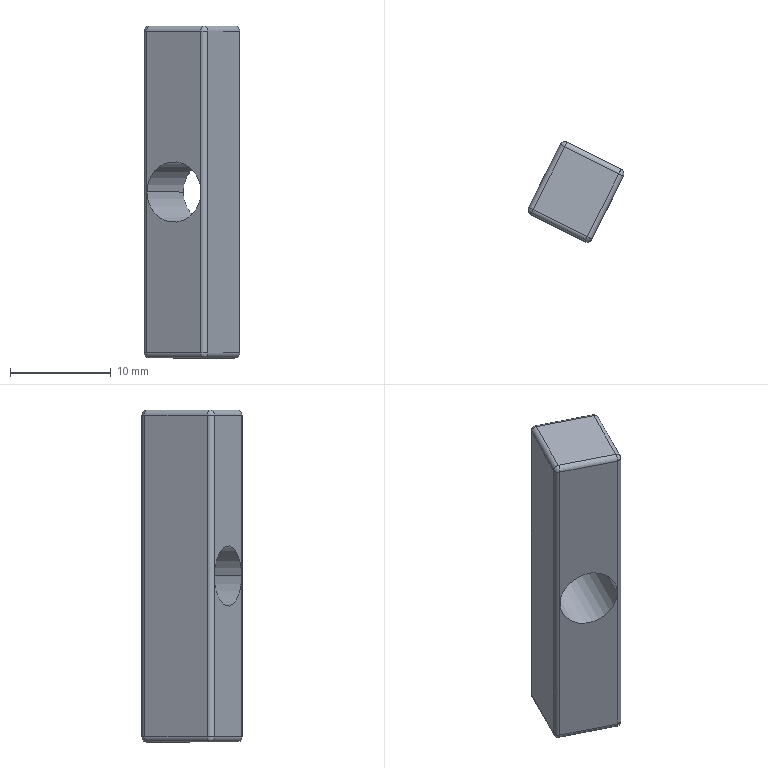Component | SolidWorks | ConnectingBlock1-1 | 1 solid | 29 faces | box 9.52 x 9.96 x 33 mm | volume 1616 mm3 | cylinder 15 | sphere 8 | plane 6 | commonest cylinder face diameters 1 x13 6 x2
STEP:
#1=CARTESIAN_POINT('',(0.6164,1.858,0.6693));
#2=VERTEX_POINT('',#1);
#3=CARTESIAN_POINT('',(0.6283,1.868,0.6693));
#4=VERTEX_POINT('',#3);
#5=CARTESIAN_POINT('',(0.634,1.849,0.6693));
#6=DIRECTION('',(-0.,-0.,-1.));
#7=DIRECTION('',(-0.2912,0.9567,0.));
#8=AXIS2_PLACEMENT_3D('',#5,#6,#7);
#9=CIRCLE('',#8,0.01969);
#10=EDGE_CURVE('',#2,#4,#9,.T.);
#11=ORIENTED_EDGE('',*,*,#10,.T.);
#12=CARTESIAN_POINT('',(0.6283,1.868,-0.5906));
#13=VERTEX_POINT('',#12);
#14=CARTESIAN_POINT('',(0.6283,1.868,0.4921));
#15=DIRECTION('',(-0.,-0.,-1.));
#16=VECTOR('',#15,39.37);
#17=LINE('',#14,#16);
#18=EDGE_CURVE('',#4,#13,#17,.T.);
#19=ORIENTED_EDGE('',*,*,#18,.T.);
#20=CARTESIAN_POINT('',(0.6164,1.858,-0.5906));
#21=VERTEX_POINT('',#20);
#22=CARTESIAN_POINT('',(0.634,1.849,-0.5906));
#23=DIRECTION('',(0.,0.,1.));
#24=DIRECTION('',(-0.2912,0.9567,0.));
#25=AXIS2_PLACEMENT_3D('',#22,#23,#24);
#26=CIRCLE('',#25,0.01969);
#27=EDGE_CURVE('',#13,#21,#26,.T.);
#28=ORIENTED_EDGE('',*,*,#27,.T.);
#29=CARTESIAN_POINT('',(0.6164,1.858,-0.6102));
#30=DIRECTION('',(-0.,-0.,-1.));
#31=VECTOR('',#30,39.37);
#32=LINE('',#29,#31);
#33=EDGE_CURVE('',#2,#21,#32,.T.);
#34=ORIENTED_EDGE('',*,*,#33,.F.);
#35=EDGE_LOOP('',(#11,#19,#28,#34));
#36=FACE_OUTER_BOUND('',#35,.T.);
#37=CARTESIAN_POINT('',(0.634,1.849,0.4921));
#38=DIRECTION('',(-0.,-0.,-1.));
#39=DIRECTION('',(-0.2912,0.9567,0.));
#40=AXIS2_PLACEMENT_3D('',#37,#38,#39);
#41=CYLINDRICAL_SURFACE('',#40,0.01969);
#42=ADVANCED_FACE('',(#36),#41,.T.);
#43=CARTESIAN_POINT('',(0.7128,1.479,0.03649));
#44=VERTEX_POINT('',#43);
#45=CARTESIAN_POINT('',(0.7128,1.479,0.03937));
#46=VERTEX_POINT('',#45);
#47=CARTESIAN_POINT('',(0.7128,1.479,0.03649));
#48=CARTESIAN_POINT('',(0.7128,1.479,0.03745));
#49=CARTESIAN_POINT('',(0.7128,1.479,0.03841));
#50=CARTESIAN_POINT('',(0.7128,1.479,0.03937));
#51=B_SPLINE_CURVE_WITH_KNOTS('',3,(#47,#48,#49,#50),.UNSPECIFIED.,.F.,.F.,(4,4),(0.,0.5),.UNSPECIFIED.);
#52=EDGE_CURVE('',#44,#46,#51,.T.);
#53=ORIENTED_EDGE('',*,*,#52,.T.);
#54=CARTESIAN_POINT('',(0.8544,1.76,0.03937));
#55=VERTEX_POINT('',#54);
#56=CARTESIAN_POINT('',(-0.3929,-0.7183,0.03937));
#57=DIRECTION('',(0.4496,0.8932,-0.));
#58=VECTOR('',#57,39.37);
#59=LINE('',#56,#58);
#60=EDGE_CURVE('',#46,#55,#59,.T.);
#61=ORIENTED_EDGE('',*,*,#60,.T.);
#62=CARTESIAN_POINT('',(0.8544,1.76,0.03649));
#63=VERTEX_POINT('',#62);
#64=CARTESIAN_POINT('',(0.8544,1.76,0.03937));
#65=CARTESIAN_POINT('',(0.8544,1.76,0.03841));
#66=CARTESIAN_POINT('',(0.8544,1.76,0.03745));
#67=CARTESIAN_POINT('',(0.8544,1.76,0.03649));
#68=B_SPLINE_CURVE_WITH_KNOTS('',3,(#64,#65,#66,#67),.UNSPECIFIED.,.F.,.F.,(4,4),(0.5,1.),.UNSPECIFIED.);
#69=EDGE_CURVE('',#55,#63,#68,.T.);
#70=ORIENTED_EDGE('',*,*,#69,.T.);
#71=CARTESIAN_POINT('',(0.6434,1.866,0.03937));
#72=VERTEX_POINT('',#71);
#73=CARTESIAN_POINT('',(0.7489,1.813,0.03937));
#74=DIRECTION('',(0.4496,0.8932,-0.));
#75=DIRECTION('',(-0.8932,0.4496,0.));
#76=AXIS2_PLACEMENT_3D('',#73,#74,#75);
#77=CIRCLE('',#76,0.1181);
#78=EDGE_CURVE('',#63,#72,#77,.T.);
#79=ORIENTED_EDGE('',*,*,#78,.T.);
#80=CARTESIAN_POINT('',(0.5018,1.585,0.03937));
#81=VERTEX_POINT('',#80);
#82=CARTESIAN_POINT('',(-0.6039,-0.6121,0.03937));
#83=DIRECTION('',(0.4496,0.8932,-0.));
#84=VECTOR('',#83,39.37);
#85=LINE('',#82,#84);
#86=EDGE_CURVE('',#81,#72,#85,.T.);
#87=ORIENTED_EDGE('',*,*,#86,.F.);
#88=CARTESIAN_POINT('',(0.6073,1.532,0.03937));
#89=DIRECTION('',(0.4496,0.8932,-0.));
#90=DIRECTION('',(-0.8932,0.4496,0.));
#91=AXIS2_PLACEMENT_3D('',#88,#89,#90);
#92=CIRCLE('',#91,0.1181);
#93=EDGE_CURVE('',#44,#81,#92,.T.);
#94=ORIENTED_EDGE('',*,*,#93,.F.);
#95=EDGE_LOOP('',(#53,#61,#70,#79,#87,#94));
#96=FACE_OUTER_BOUND('',#95,.T.);
#97=CARTESIAN_POINT('',(-0.4984,-0.6652,0.03937));
#98=DIRECTION('',(0.4496,0.8932,-0.));
#99=DIRECTION('',(-0.8932,0.4496,0.));
#100=AXIS2_PLACEMENT_3D('',#97,#98,#99);
#101=CYLINDRICAL_SURFACE('',#100,0.1181);
#102=ADVANCED_FACE('',(#96),#101,.F.);
#103=ORIENTED_EDGE('',*,*,#60,.F.);
#104=CARTESIAN_POINT('',(0.7128,1.479,0.04225));
#105=VERTEX_POINT('',#104);
#106=CARTESIAN_POINT('',(0.7128,1.479,0.03937));
#107=CARTESIAN_POINT('',(0.7128,1.479,0.04033));
#108=CARTESIAN_POINT('',(0.7128,1.479,0.04129));
#109=CARTESIAN_POINT('',(0.7128,1.479,0.04225));
#110=B_SPLINE_CURVE_WITH_KNOTS('',3,(#106,#107,#108,#109),.UNSPECIFIED.,.F.,.F.,(4,4),(0.5,1.),.UNSPECIFIED.);
#111=EDGE_CURVE('',#46,#105,#110,.T.);
#112=ORIENTED_EDGE('',*,*,#111,.T.);
#113=CARTESIAN_POINT('',(0.6073,1.532,0.03937));
#114=DIRECTION('',(0.4496,0.8932,-0.));
#115=DIRECTION('',(-0.8932,0.4496,0.));
#116=AXIS2_PLACEMENT_3D('',#113,#114,#115);
#117=CIRCLE('',#116,0.1181);
#118=EDGE_CURVE('',#81,#105,#117,.T.);
#119=ORIENTED_EDGE('',*,*,#118,.F.);
#120=ORIENTED_EDGE('',*,*,#86,.T.);
#121=CARTESIAN_POINT('',(0.8544,1.76,0.04225));
#122=VERTEX_POINT('',#121);
#123=CARTESIAN_POINT('',(0.7489,1.813,0.03937));
#124=DIRECTION('',(0.4496,0.8932,-0.));
#125=DIRECTION('',(-0.8932,0.4496,0.));
#126=AXIS2_PLACEMENT_3D('',#123,#124,#125);
#127=CIRCLE('',#126,0.1181);
#128=EDGE_CURVE('',#72,#122,#127,.T.);
#129=ORIENTED_EDGE('',*,*,#128,.T.);
#130=CARTESIAN_POINT('',(0.8544,1.76,0.04225));
#131=CARTESIAN_POINT('',(0.8544,1.76,0.04129));
#132=CARTESIAN_POINT('',(0.8544,1.76,0.04033));
#133=CARTESIAN_POINT('',(0.8544,1.76,0.03937));
#134=B_SPLINE_CURVE_WITH_KNOTS('',3,(#130,#131,#132,#133),.UNSPECIFIED.,.F.,.F.,(4,4),(0.,0.5),.UNSPECIFIED.);
#135=EDGE_CURVE('',#122,#55,#134,.T.);
#136=ORIENTED_EDGE('',*,*,#135,.T.);
#137=EDGE_LOOP('',(#103,#112,#119,#120,#129,#136));
#138=FACE_OUTER_BOUND('',#137,.T.);
#139=CARTESIAN_POINT('',(-0.4984,-0.6652,0.03937));
#140=DIRECTION('',(0.4496,0.8932,-0.));
#141=DIRECTION('',(-0.8932,0.4496,0.));
#142=AXIS2_PLACEMENT_3D('',#139,#140,#141);
#143=CYLINDRICAL_SURFACE('',#142,0.1181);
#144=ADVANCED_FACE('',(#138),#143,.F.);
#145=CARTESIAN_POINT('',(0.7128,1.479,-0.5906));
#146=VERTEX_POINT('',#145);
#147=CARTESIAN_POINT('',(0.7216,1.496,-0.6102));
#148=VERTEX_POINT('',#147);
#149=CARTESIAN_POINT('',(0.7216,1.496,-0.5906));
#150=DIRECTION('',(0.8932,-0.4496,-0.));
#151=DIRECTION('',(0.4496,0.8932,0.));
#152=AXIS2_PLACEMENT_3D('',#149,#150,#151);
#153=CIRCLE('',#152,0.01969);
#154=EDGE_CURVE('',#146,#148,#153,.T.);
#155=ORIENTED_EDGE('',*,*,#154,.T.);
#156=CARTESIAN_POINT('',(0.7392,1.487,-0.5906));
#157=VERTEX_POINT('',#156);
#158=CARTESIAN_POINT('',(0.7216,1.496,-0.5906));
#159=DIRECTION('',(0.4496,0.8932,-0.));
#160=DIRECTION('',(0.8932,-0.4496,0.));
#161=AXIS2_PLACEMENT_3D('',#158,#159,#160);
#162=CIRCLE('',#161,0.01969);
#163=EDGE_CURVE('',#157,#148,#162,.T.);
#164=ORIENTED_EDGE('',*,*,#163,.F.);
#165=CARTESIAN_POINT('',(0.7216,1.496,-0.5906));
#166=DIRECTION('',(0.,0.,1.));
#167=DIRECTION('',(-0.2912,0.9567,0.));
#168=AXIS2_PLACEMENT_3D('',#165,#166,#167);
#169=CIRCLE('',#168,0.01969);
#170=EDGE_CURVE('',#146,#157,#169,.T.);
#171=ORIENTED_EDGE('',*,*,#170,.F.);
#172=EDGE_LOOP('',(#155,#164,#171));
#173=FACE_OUTER_BOUND('',#172,.T.);
#174=CARTESIAN_POINT('',(0.7216,1.496,-0.5906));
#175=DIRECTION('',(0.,-0.,-1.));
#176=DIRECTION('',(0.9567,0.2912,0.));
#177=AXIS2_PLACEMENT_3D('',#174,#175,#176);
#178=SPHERICAL_SURFACE('',#177,0.01969);
#179=ADVANCED_FACE('',(#173),#178,.T.);
#180=CARTESIAN_POINT('',(0.5012,1.585,-0.5906));
#181=VERTEX_POINT('',#180);
#182=CARTESIAN_POINT('',(0.5101,1.603,-0.6102));
#183=VERTEX_POINT('',#182);
#184=CARTESIAN_POINT('',(0.5101,1.603,-0.5906));
#185=DIRECTION('',(0.8932,-0.4496,-0.));
#186=DIRECTION('',(0.4496,0.8932,0.));
#187=AXIS2_PLACEMENT_3D('',#184,#185,#186);
#188=CIRCLE('',#187,0.01969);
#189=EDGE_CURVE('',#181,#183,#188,.T.);
#190=ORIENTED_EDGE('',*,*,#189,.T.);
#191=CARTESIAN_POINT('',(0.4925,1.612,-0.6102));
#192=DIRECTION('',(-0.8932,0.4496,0.));
#193=VECTOR('',#192,39.37);
#194=LINE('',#191,#193);
#195=EDGE_CURVE('',#148,#183,#194,.T.);
#196=ORIENTED_EDGE('',*,*,#195,.F.);
#197=ORIENTED_EDGE('',*,*,#154,.F.);
#198=CARTESIAN_POINT('',(0.5768,1.547,-0.5906));
#199=DIRECTION('',(0.8932,-0.4496,-0.));
#200=VECTOR('',#199,39.37);
#201=LINE('',#198,#200);
#202=EDGE_CURVE('',#181,#146,#201,.T.);
#203=ORIENTED_EDGE('',*,*,#202,.F.);
#204=EDGE_LOOP('',(#190,#196,#197,#203));
#205=FACE_OUTER_BOUND('',#204,.T.);
#206=CARTESIAN_POINT('',(0.4925,1.612,-0.5906));
#207=DIRECTION('',(-0.8932,0.4496,0.));
#208=DIRECTION('',(-0.4496,-0.8932,0.));
#209=AXIS2_PLACEMENT_3D('',#206,#207,#208);
#210=CYLINDRICAL_SURFACE('',#209,0.01969);
#211=ADVANCED_FACE('',(#205),#210,.T.);
#212=CARTESIAN_POINT('',(0.4925,1.612,-0.5906));
#213=VERTEX_POINT('',#212);
#214=CARTESIAN_POINT('',(0.5101,1.603,-0.5906));
#215=DIRECTION('',(0.,0.,1.));
#216=DIRECTION('',(0.2912,-0.9567,0.));
#217=AXIS2_PLACEMENT_3D('',#214,#215,#216);
#218=CIRCLE('',#217,0.01969);
#219=EDGE_CURVE('',#213,#181,#218,.T.);
#220=ORIENTED_EDGE('',*,*,#219,.F.);
#221=CARTESIAN_POINT('',(0.5101,1.603,-0.5906));
#222=DIRECTION('',(0.4496,0.8932,-0.));
#223=DIRECTION('',(0.8932,-0.4496,0.));
#224=AXIS2_PLACEMENT_3D('',#221,#222,#223);
#225=CIRCLE('',#224,0.01969);
#226=EDGE_CURVE('',#183,#213,#225,.T.);
#227=ORIENTED_EDGE('',*,*,#226,.F.);
#228=ORIENTED_EDGE('',*,*,#189,.F.);
#229=EDGE_LOOP('',(#220,#227,#228));
#230=FACE_OUTER_BOUND('',#229,.T.);
#231=CARTESIAN_POINT('',(0.5101,1.603,-0.5906));
#232=DIRECTION('',(0.,-0.,-1.));
#233=DIRECTION('',(0.9567,0.2912,0.));
#234=AXIS2_PLACEMENT_3D('',#231,#232,#233);
#235=SPHERICAL_SURFACE('',#234,0.01969);
#236=ADVANCED_FACE('',(#230),#235,.T.);
#237=CARTESIAN_POINT('',(0.5012,1.585,0.6693));
#238=VERTEX_POINT('',#237);
#239=CARTESIAN_POINT('',(0.5101,1.603,0.689));
#240=VERTEX_POINT('',#239);
#241=CARTESIAN_POINT('',(0.5101,1.603,0.6693));
#242=DIRECTION('',(-0.8932,0.4496,0.));
#243=DIRECTION('',(-0.4496,-0.8932,0.));
#244=AXIS2_PLACEMENT_3D('',#241,#242,#243);
#245=CIRCLE('',#244,0.01969);
#246=EDGE_CURVE('',#238,#240,#245,.T.);
#247=ORIENTED_EDGE('',*,*,#246,.T.);
#248=CARTESIAN_POINT('',(0.4925,1.612,0.6693));
#249=VERTEX_POINT('',#248);
#250=CARTESIAN_POINT('',(0.5101,1.603,0.6693));
#251=DIRECTION('',(0.4496,0.8932,-0.));
#252=DIRECTION('',(0.8932,-0.4496,0.));
#253=AXIS2_PLACEMENT_3D('',#250,#251,#252);
#254=CIRCLE('',#253,0.01969);
#255=EDGE_CURVE('',#249,#240,#254,.T.);
#256=ORIENTED_EDGE('',*,*,#255,.F.);
#257=CARTESIAN_POINT('',(0.5101,1.603,0.6693));
#258=DIRECTION('',(-0.,-0.,-1.));
#259=DIRECTION('',(0.2912,-0.9567,0.));
#260=AXIS2_PLACEMENT_3D('',#257,#258,#259);
#261=CIRCLE('',#260,0.01969);
#262=EDGE_CURVE('',#238,#249,#261,.T.);
#263=ORIENTED_EDGE('',*,*,#262,.F.);
#264=EDGE_LOOP('',(#247,#256,#263));
#265=FACE_OUTER_BOUND('',#264,.T.);
#266=CARTESIAN_POINT('',(0.5101,1.603,0.6693));
#267=DIRECTION('',(0.,-0.,-1.));
#268=DIRECTION('',(0.9567,0.2912,0.));
#269=AXIS2_PLACEMENT_3D('',#266,#267,#268);
#270=SPHERICAL_SURFACE('',#269,0.01969);
#271=ADVANCED_FACE('',(#265),#270,.T.);
#272=CARTESIAN_POINT('',(0.7128,1.479,0.6693));
#273=VERTEX_POINT('',#272);
#274=CARTESIAN_POINT('',(0.7216,1.496,0.689));
#275=VERTEX_POINT('',#274);
#276=CARTESIAN_POINT('',(0.7216,1.496,0.6693));
#277=DIRECTION('',(-0.8932,0.4496,0.));
#278=DIRECTION('',(-0.4496,-0.8932,0.));
#279=AXIS2_PLACEMENT_3D('',#276,#277,#278);
#280=CIRCLE('',#279,0.01969);
#281=EDGE_CURVE('',#273,#275,#280,.T.);
#282=ORIENTED_EDGE('',*,*,#281,.T.);
#283=CARTESIAN_POINT('',(0.4925,1.612,0.689));
#284=DIRECTION('',(0.8932,-0.4496,-0.));
#285=VECTOR('',#284,39.37);
#286=LINE('',#283,#285);
#287=EDGE_CURVE('',#240,#275,#286,.T.);
#288=ORIENTED_EDGE('',*,*,#287,.F.);
#289=ORIENTED_EDGE('',*,*,#246,.F.);
#290=CARTESIAN_POINT('',(0.5768,1.547,0.6693));
#291=DIRECTION('',(-0.8932,0.4496,0.));
#292=VECTOR('',#291,39.37);
#293=LINE('',#290,#292);
#294=EDGE_CURVE('',#273,#238,#293,.T.);
#295=ORIENTED_EDGE('',*,*,#294,.F.);
#296=EDGE_LOOP('',(#282,#288,#289,#295));
#297=FACE_OUTER_BOUND('',#296,.T.);
#298=CARTESIAN_POINT('',(0.4925,1.612,0.6693));
#299=DIRECTION('',(0.8932,-0.4496,-0.));
#300=DIRECTION('',(0.4496,0.8932,0.));
#301=AXIS2_PLACEMENT_3D('',#298,#299,#300);
#302=CYLINDRICAL_SURFACE('',#301,0.01969);
#303=ADVANCED_FACE('',(#297),#302,.T.);
#304=CARTESIAN_POINT('',(0.7392,1.487,0.6693));
#305=VERTEX_POINT('',#304);
#306=CARTESIAN_POINT('',(0.7216,1.496,0.6693));
#307=DIRECTION('',(-0.,-0.,-1.));
#308=DIRECTION('',(-0.2912,0.9567,0.));
#309=AXIS2_PLACEMENT_3D('',#306,#307,#308);
#310=CIRCLE('',#309,0.01969);
#311=EDGE_CURVE('',#305,#273,#310,.T.);
#312=ORIENTED_EDGE('',*,*,#311,.F.);
#313=CARTESIAN_POINT('',(0.7216,1.496,0.6693));
#314=DIRECTION('',(0.4496,0.8932,-0.));
#315=DIRECTION('',(0.8932,-0.4496,-0.));
#316=AXIS2_PLACEMENT_3D('',#313,#314,#315);
#317=CIRCLE('',#316,0.01969);
#318=EDGE_CURVE('',#275,#305,#317,.T.);
#319=ORIENTED_EDGE('',*,*,#318,.F.);
#320=ORIENTED_EDGE('',*,*,#281,.F.);
#321=EDGE_LOOP('',(#312,#319,#320));
#322=FACE_OUTER_BOUND('',#321,.T.);
#323=CARTESIAN_POINT('',(0.7216,1.496,0.6693));
#324=DIRECTION('',(0.,-0.,-1.));
#325=DIRECTION('',(0.9567,0.2912,0.));
#326=AXIS2_PLACEMENT_3D('',#323,#324,#325);
#327=SPHERICAL_SURFACE('',#326,0.01969);
#328=ADVANCED_FACE('',(#322),#327,.T.);
#329=ORIENTED_EDGE('',*,*,#10,.F.);
#330=CARTESIAN_POINT('',(0.634,1.849,0.689));
#331=VERTEX_POINT('',#330);
#332=CARTESIAN_POINT('',(0.634,1.849,0.6693));
#333=DIRECTION('',(-0.4496,-0.8932,0.));
#334=DIRECTION('',(0.8932,-0.4496,0.));
#335=AXIS2_PLACEMENT_3D('',#332,#333,#334);
#336=CIRCLE('',#335,0.01969);
#337=EDGE_CURVE('',#331,#2,#336,.T.);
#338=ORIENTED_EDGE('',*,*,#337,.F.);
#339=CARTESIAN_POINT('',(0.6428,1.866,0.6693));
#340=VERTEX_POINT('',#339);
#341=CARTESIAN_POINT('',(0.634,1.849,0.6693));
#342=DIRECTION('',(-0.8932,0.4496,0.));
#343=DIRECTION('',(-0.4496,-0.8932,0.));
#344=AXIS2_PLACEMENT_3D('',#341,#342,#343);
#345=CIRCLE('',#344,0.01969);
#346=EDGE_CURVE('',#331,#340,#345,.T.);
#347=ORIENTED_EDGE('',*,*,#346,.T.);
#348=CARTESIAN_POINT('',(0.634,1.849,0.6693));
#349=DIRECTION('',(-0.,-0.,-1.));
#350=DIRECTION('',(-0.2912,0.9567,0.));
#351=AXIS2_PLACEMENT_3D('',#348,#349,#350);
#352=CIRCLE('',#351,0.01969);
#353=EDGE_CURVE('',#4,#340,#352,.T.);
#354=ORIENTED_EDGE('',*,*,#353,.F.);
#355=EDGE_LOOP('',(#329,#338,#347,#354));
#356=FACE_OUTER_BOUND('',#355,.T.);
#357=CARTESIAN_POINT('',(0.634,1.849,0.6693));
#358=DIRECTION('',(0.,-0.,-1.));
#359=DIRECTION('',(0.9567,0.2912,0.));
#360=AXIS2_PLACEMENT_3D('',#357,#358,#359);
#361=SPHERICAL_SURFACE('',#360,0.01969);
#362=ADVANCED_FACE('',(#356),#361,.T.);
#363=CARTESIAN_POINT('',(0.8455,1.742,0.689));
#364=VERTEX_POINT('',#363);
#365=CARTESIAN_POINT('',(0.8544,1.76,0.6693));
#366=VERTEX_POINT('',#365);
#367=CARTESIAN_POINT('',(0.8455,1.742,0.6693));
#368=DIRECTION('',(-0.8932,0.4496,0.));
#369=DIRECTION('',(-0.4496,-0.8932,0.));
#370=AXIS2_PLACEMENT_3D('',#367,#368,#369);
#371=CIRCLE('',#370,0.01969);
#372=EDGE_CURVE('',#364,#366,#371,.T.);
#373=ORIENTED_EDGE('',*,*,#372,.T.);
#374=CARTESIAN_POINT('',(0.8544,1.76,0.6693));
#375=DIRECTION('',(0.8932,-0.4496,-0.));
#376=VECTOR('',#375,39.37);
#377=LINE('',#374,#376);
#378=EDGE_CURVE('',#340,#366,#377,.T.);
#379=ORIENTED_EDGE('',*,*,#378,.F.);
#380=ORIENTED_EDGE('',*,*,#346,.F.);
#381=CARTESIAN_POINT('',(0.634,1.849,0.689));
#382=DIRECTION('',(-0.8932,0.4496,0.));
#383=VECTOR('',#382,39.37);
#384=LINE('',#381,#383);
#385=EDGE_CURVE('',#364,#331,#384,.T.);
#386=ORIENTED_EDGE('',*,*,#385,.F.);
#387=EDGE_LOOP('',(#373,#379,#380,#386));
#388=FACE_OUTER_BOUND('',#387,.T.);
#389=CARTESIAN_POINT('',(0.7095,1.811,0.6693));
#390=DIRECTION('',(-0.8932,0.4496,0.));
#391=DIRECTION('',(-0.4496,-0.8932,0.));
#392=AXIS2_PLACEMENT_3D('',#389,#390,#391);
#393=CYLINDRICAL_SURFACE('',#392,0.01969);
#394=ADVANCED_FACE('',(#388),#393,.T.);
#395=CARTESIAN_POINT('',(0.8631,1.734,0.6693));
#396=VERTEX_POINT('',#395);
#397=CARTESIAN_POINT('',(0.8455,1.742,0.6693));
#398=DIRECTION('',(-0.4496,-0.8932,0.));
#399=DIRECTION('',(0.8932,-0.4496,0.));
#400=AXIS2_PLACEMENT_3D('',#397,#398,#399);
#401=CIRCLE('',#400,0.01969);
#402=EDGE_CURVE('',#396,#364,#401,.T.);
#403=ORIENTED_EDGE('',*,*,#402,.F.);
#404=CARTESIAN_POINT('',(0.8455,1.742,0.6693));
#405=DIRECTION('',(-0.,-0.,-1.));
#406=DIRECTION('',(0.2912,-0.9567,0.));
#407=AXIS2_PLACEMENT_3D('',#404,#405,#406);
#408=CIRCLE('',#407,0.01969);
#409=EDGE_CURVE('',#366,#396,#408,.T.);
#410=ORIENTED_EDGE('',*,*,#409,.F.);
#411=ORIENTED_EDGE('',*,*,#372,.F.);
#412=EDGE_LOOP('',(#403,#410,#411));
#413=FACE_OUTER_BOUND('',#412,.T.);
#414=CARTESIAN_POINT('',(0.8455,1.742,0.6693));
#415=DIRECTION('',(0.,-0.,-1.));
#416=DIRECTION('',(0.9567,0.2912,0.));
#417=AXIS2_PLACEMENT_3D('',#414,#415,#416);
#418=SPHERICAL_SURFACE('',#417,0.01969);
#419=ADVANCED_FACE('',(#413),#418,.T.);
#420=CARTESIAN_POINT('',(0.8631,1.734,-0.5906));
#421=VERTEX_POINT('',#420);
#422=CARTESIAN_POINT('',(0.8544,1.76,-0.5906));
#423=VERTEX_POINT('',#422);
#424=CARTESIAN_POINT('',(0.8455,1.742,-0.5906));
#425=DIRECTION('',(0.,0.,1.));
#426=DIRECTION('',(0.2912,-0.9567,0.));
#427=AXIS2_PLACEMENT_3D('',#424,#425,#426);
#428=CIRCLE('',#427,0.01969);
#429=EDGE_CURVE('',#421,#423,#428,.T.);
#430=ORIENTED_EDGE('',*,*,#429,.F.);
#431=CARTESIAN_POINT('',(0.8455,1.742,-0.6102));
#432=VERTEX_POINT('',#431);
#433=CARTESIAN_POINT('',(0.8455,1.742,-0.5906));
#434=DIRECTION('',(-0.4496,-0.8932,0.));
#435=DIRECTION('',(0.8932,-0.4496,0.));
#436=AXIS2_PLACEMENT_3D('',#433,#434,#435);
#437=CIRCLE('',#436,0.01969);
#438=EDGE_CURVE('',#432,#421,#437,.T.);
#439=ORIENTED_EDGE('',*,*,#438,.F.);
#440=CARTESIAN_POINT('',(0.8455,1.742,-0.5906));
#441=DIRECTION('',(0.8932,-0.4496,-0.));
#442=DIRECTION('',(0.4496,0.8932,0.));
#443=AXIS2_PLACEMENT_3D('',#440,#441,#442);
#444=CIRCLE('',#443,0.01969);
#445=EDGE_CURVE('',#432,#423,#444,.T.);
#446=ORIENTED_EDGE('',*,*,#445,.T.);
#447=EDGE_LOOP('',(#430,#439,#446));
#448=FACE_OUTER_BOUND('',#447,.T.);
#449=CARTESIAN_POINT('',(0.8455,1.742,-0.5906));
#450=DIRECTION('',(0.,-0.,-1.));
#451=DIRECTION('',(0.9567,0.2912,0.));
#452=AXIS2_PLACEMENT_3D('',#449,#450,#451);
#453=SPHERICAL_SURFACE('',#452,0.01969);
#454=ADVANCED_FACE('',(#448),#453,.T.);
#455=CARTESIAN_POINT('',(0.634,1.849,-0.6102));
#456=VERTEX_POINT('',#455);
#457=CARTESIAN_POINT('',(0.6428,1.866,-0.5906));
#458=VERTEX_POINT('',#457);
#459=CARTESIAN_POINT('',(0.634,1.849,-0.5906));
#460=DIRECTION('',(0.8932,-0.4496,-0.));
#461=DIRECTION('',(0.4496,0.8932,0.));
#462=AXIS2_PLACEMENT_3D('',#459,#460,#461);
#463=CIRCLE('',#462,0.01969);
#464=EDGE_CURVE('',#456,#458,#463,.T.);
#465=ORIENTED_EDGE('',*,*,#464,.T.);
#466=CARTESIAN_POINT('',(0.6428,1.866,-0.5906));
#467=DIRECTION('',(-0.8932,0.4496,0.));
#468=VECTOR('',#467,39.37);
#469=LINE('',#466,#468);
#470=EDGE_CURVE('',#423,#458,#469,.T.);
#471=ORIENTED_EDGE('',*,*,#470,.F.);
#472=ORIENTED_EDGE('',*,*,#445,.F.);
#473=CARTESIAN_POINT('',(0.8455,1.742,-0.6102));
#474=DIRECTION('',(0.8932,-0.4496,-0.));
#475=VECTOR('',#474,39.37);
#476=LINE('',#473,#475);
#477=EDGE_CURVE('',#456,#432,#476,.T.);
#478=ORIENTED_EDGE('',*,*,#477,.F.);
#479=EDGE_LOOP('',(#465,#471,#472,#478));
#480=FACE_OUTER_BOUND('',#479,.T.);
#481=CARTESIAN_POINT('',(0.7095,1.811,-0.5906));
#482=DIRECTION('',(0.8932,-0.4496,-0.));
#483=DIRECTION('',(0.4496,0.8932,0.));
#484=AXIS2_PLACEMENT_3D('',#481,#482,#483);
#485=CYLINDRICAL_SURFACE('',#484,0.01969);
#486=ADVANCED_FACE('',(#480),#485,.T.);
#487=CARTESIAN_POINT('',(0.634,1.849,-0.5906));
#488=DIRECTION('',(-0.4496,-0.8932,0.));
#489=DIRECTION('',(0.8932,-0.4496,0.));
#490=AXIS2_PLACEMENT_3D('',#487,#488,#489);
#491=CIRCLE('',#490,0.01969);
#492=EDGE_CURVE('',#21,#456,#491,.T.);
#493=ORIENTED_EDGE('',*,*,#492,.F.);
#494=ORIENTED_EDGE('',*,*,#27,.F.);
#495=CARTESIAN_POINT('',(0.634,1.849,-0.5906));
#496=DIRECTION('',(0.,0.,1.));
#497=DIRECTION('',(-0.2912,0.9567,0.));
#498=AXIS2_PLACEMENT_3D('',#495,#496,#497);
#499=CIRCLE('',#498,0.01969);
#500=EDGE_CURVE('',#458,#13,#499,.T.);
#501=ORIENTED_EDGE('',*,*,#500,.F.);
#502=ORIENTED_EDGE('',*,*,#464,.F.);
#503=EDGE_LOOP('',(#493,#494,#501,#502));
#504=FACE_OUTER_BOUND('',#503,.T.);
#505=CARTESIAN_POINT('',(0.634,1.849,-0.5906));
#506=DIRECTION('',(0.,-0.,-1.));
#507=DIRECTION('',(0.9567,0.2912,0.));
#508=AXIS2_PLACEMENT_3D('',#505,#506,#507);
#509=SPHERICAL_SURFACE('',#508,0.01969);
#510=ADVANCED_FACE('',(#504),#509,.T.);
#511=CARTESIAN_POINT('',(0.6253,1.875,-0.5906));
#512=DIRECTION('',(-0.4496,-0.8932,0.));
#513=VECTOR('',#512,39.37);
#514=LINE('',#511,#513);
#515=EDGE_CURVE('',#21,#213,#514,.T.);
#516=ORIENTED_EDGE('',*,*,#515,.F.);
#517=ORIENTED_EDGE('',*,*,#492,.T.);
#518=CARTESIAN_POINT('',(0.6428,1.866,-0.6102));
#519=DIRECTION('',(0.4496,0.8932,-0.));
#520=VECTOR('',#519,39.37);
#521=LINE('',#518,#520);
#522=EDGE_CURVE('',#183,#456,#521,.T.);
#523=ORIENTED_EDGE('',*,*,#522,.F.);
#524=ORIENTED_EDGE('',*,*,#226,.T.);
#525=EDGE_LOOP('',(#516,#517,#523,#524));
#526=FACE_OUTER_BOUND('',#525,.T.);
#527=CARTESIAN_POINT('',(0.6428,1.866,-0.5906));
#528=DIRECTION('',(-0.4496,-0.8932,0.));
#529=DIRECTION('',(0.8932,-0.4496,0.));
#530=AXIS2_PLACEMENT_3D('',#527,#528,#529);
#531=CYLINDRICAL_SURFACE('',#530,0.01969);
#532=ADVANCED_FACE('',(#526),#531,.T.);
#533=CARTESIAN_POINT('',(0.5012,1.585,0.4921));
#534=DIRECTION('',(-0.,-0.,-1.));
#535=VECTOR('',#534,39.37);
#536=LINE('',#533,#535);
#537=EDGE_CURVE('',#238,#181,#536,.T.);
#538=ORIENTED_EDGE('',*,*,#537,.F.);
#539=ORIENTED_EDGE('',*,*,#262,.T.);
#540=CARTESIAN_POINT('',(0.4925,1.612,-0.6102));
#541=DIRECTION('',(0.,0.,1.));
#542=VECTOR('',#541,39.37);
#543=LINE('',#540,#542);
#544=EDGE_CURVE('',#213,#249,#543,.T.);
#545=ORIENTED_EDGE('',*,*,#544,.F.);
#546=ORIENTED_EDGE('',*,*,#219,.T.);
#547=EDGE_LOOP('',(#538,#539,#545,#546));
#548=FACE_OUTER_BOUND('',#547,.T.);
#549=CARTESIAN_POINT('',(0.5101,1.603,-0.6102));
#550=DIRECTION('',(0.,0.,1.));
#551=DIRECTION('',(0.2912,-0.9567,0.));
#552=AXIS2_PLACEMENT_3D('',#549,#550,#551);
#553=CYLINDRICAL_SURFACE('',#552,0.01969);
#554=ADVANCED_FACE('',(#548),#553,.T.);
#555=ORIENTED_EDGE('',*,*,#18,.F.);
#556=ORIENTED_EDGE('',*,*,#353,.T.);
#557=CARTESIAN_POINT('',(0.6428,1.866,0.689));
#558=DIRECTION('',(0.,0.,1.));
#559=VECTOR('',#558,39.37);
#560=LINE('',#557,#559);
#561=EDGE_CURVE('',#458,#340,#560,.T.);
#562=ORIENTED_EDGE('',*,*,#561,.F.);
#563=ORIENTED_EDGE('',*,*,#500,.T.);
#564=EDGE_LOOP('',(#555,#556,#562,#563));
#565=FACE_OUTER_BOUND('',#564,.T.);
#566=CARTESIAN_POINT('',(0.634,1.849,0.4921));
#567=DIRECTION('',(-0.,-0.,-1.));
#568=DIRECTION('',(-0.2912,0.9567,0.));
#569=AXIS2_PLACEMENT_3D('',#566,#567,#568);
#570=CYLINDRICAL_SURFACE('',#569,0.01969);
#571=ADVANCED_FACE('',(#565),#570,.T.);
#572=CARTESIAN_POINT('',(0.6428,1.866,0.689));
#573=DIRECTION('',(-0.4496,-0.8932,0.));
#574=VECTOR('',#573,39.37);
#575=LINE('',#572,#574);
#576=EDGE_CURVE('',#331,#240,#575,.T.);
#577=ORIENTED_EDGE('',*,*,#576,.F.);
#578=ORIENTED_EDGE('',*,*,#337,.T.);
#579=CARTESIAN_POINT('',(0.6253,1.875,0.6693));
#580=DIRECTION('',(0.4496,0.8932,-0.));
#581=VECTOR('',#580,39.37);
#582=LINE('',#579,#581);
#583=EDGE_CURVE('',#249,#2,#582,.T.);
#584=ORIENTED_EDGE('',*,*,#583,.F.);
#585=ORIENTED_EDGE('',*,*,#255,.T.);
#586=EDGE_LOOP('',(#577,#578,#584,#585));
#587=FACE_OUTER_BOUND('',#586,.T.);
#588=CARTESIAN_POINT('',(0.6428,1.866,0.6693));
#589=DIRECTION('',(-0.4496,-0.8932,0.));
#590=DIRECTION('',(0.8932,-0.4496,0.));
#591=AXIS2_PLACEMENT_3D('',#588,#589,#590);
#592=CYLINDRICAL_SURFACE('',#591,0.01969);
#593=ADVANCED_FACE('',(#587),#592,.T.);
#594=CARTESIAN_POINT('',(0.872,1.751,0.6693));
#595=DIRECTION('',(-0.4496,-0.8932,0.));
#596=VECTOR('',#595,39.37);
#597=LINE('',#594,#596);
#598=EDGE_CURVE('',#396,#305,#597,.T.);
#599=ORIENTED_EDGE('',*,*,#598,.F.);
#600=ORIENTED_EDGE('',*,*,#402,.T.);
#601=CARTESIAN_POINT('',(0.8544,1.76,0.689));
#602=DIRECTION('',(0.4496,0.8932,-0.));
#603=VECTOR('',#602,39.37);
#604=LINE('',#601,#603);
#605=EDGE_CURVE('',#275,#364,#604,.T.);
#606=ORIENTED_EDGE('',*,*,#605,.F.);
#607=ORIENTED_EDGE('',*,*,#318,.T.);
#608=EDGE_LOOP('',(#599,#600,#606,#607));
#609=FACE_OUTER_BOUND('',#608,.T.);
#610=CARTESIAN_POINT('',(0.8544,1.76,0.6693));
#611=DIRECTION('',(-0.4496,-0.8932,0.));
#612=DIRECTION('',(0.8932,-0.4496,0.));
#613=AXIS2_PLACEMENT_3D('',#610,#611,#612);
#614=CYLINDRICAL_SURFACE('',#613,0.01969);
#615=ADVANCED_FACE('',(#609),#614,.T.);
#616=ORIENTED_EDGE('',*,*,#52,.F.);
#617=CARTESIAN_POINT('',(0.7128,1.479,0.4921));
#618=DIRECTION('',(0.,0.,1.));
#619=VECTOR('',#618,39.37);
#620=LINE('',#617,#619);
#621=EDGE_CURVE('',#146,#44,#620,.T.);
#622=ORIENTED_EDGE('',*,*,#621,.F.);
#623=ORIENTED_EDGE('',*,*,#170,.T.);
#624=CARTESIAN_POINT('',(0.7392,1.487,-0.6102));
#625=DIRECTION('',(-0.,-0.,-1.));
#626=VECTOR('',#625,39.37);
#627=LINE('',#624,#626);
#628=EDGE_CURVE('',#305,#157,#627,.T.);
#629=ORIENTED_EDGE('',*,*,#628,.F.);
#630=ORIENTED_EDGE('',*,*,#311,.T.);
#631=CARTESIAN_POINT('',(0.7128,1.479,0.4921));
#632=DIRECTION('',(0.,0.,1.));
#633=VECTOR('',#632,39.37);
#634=LINE('',#631,#633);
#635=EDGE_CURVE('',#105,#273,#634,.T.);
#636=ORIENTED_EDGE('',*,*,#635,.F.);
#637=ORIENTED_EDGE('',*,*,#111,.F.);
#638=EDGE_LOOP('',(#616,#622,#623,#629,#630,#636,#637));
#639=FACE_OUTER_BOUND('',#638,.T.);
#640=CARTESIAN_POINT('',(0.7216,1.496,-0.6102));
#641=DIRECTION('',(-0.,-0.,-1.));
#642=DIRECTION('',(-0.2912,0.9567,0.));
#643=AXIS2_PLACEMENT_3D('',#640,#641,#642);
#644=CYLINDRICAL_SURFACE('',#643,0.01969);
#645=ADVANCED_FACE('',(#639),#644,.T.);
#646=ORIENTED_EDGE('',*,*,#135,.F.);
#647=CARTESIAN_POINT('',(0.8544,1.76,-0.6102));
#648=DIRECTION('',(-0.,-0.,-1.));
#649=VECTOR('',#648,39.37);
#650=LINE('',#647,#649);
#651=EDGE_CURVE('',#366,#122,#650,.T.);
#652=ORIENTED_EDGE('',*,*,#651,.F.);
#653=ORIENTED_EDGE('',*,*,#409,.T.);
#654=CARTESIAN_POINT('',(0.8631,1.734,0.689));
#655=DIRECTION('',(0.,0.,1.));
#656=VECTOR('',#655,39.37);
#657=LINE('',#654,#656);
#658=EDGE_CURVE('',#421,#396,#657,.T.);
#659=ORIENTED_EDGE('',*,*,#658,.F.);
#660=ORIENTED_EDGE('',*,*,#429,.T.);
#661=CARTESIAN_POINT('',(0.8544,1.76,-0.6102));
#662=DIRECTION('',(-0.,-0.,-1.));
#663=VECTOR('',#662,39.37);
#664=LINE('',#661,#663);
#665=EDGE_CURVE('',#63,#423,#664,.T.);
#666=ORIENTED_EDGE('',*,*,#665,.F.);
#667=ORIENTED_EDGE('',*,*,#69,.F.);
#668=EDGE_LOOP('',(#646,#652,#653,#659,#660,#666,#667));
#669=FACE_OUTER_BOUND('',#668,.T.);
#670=CARTESIAN_POINT('',(0.8455,1.742,0.4921));
#671=DIRECTION('',(0.,0.,1.));
#672=DIRECTION('',(0.2912,-0.9567,0.));
#673=AXIS2_PLACEMENT_3D('',#670,#671,#672);
#674=CYLINDRICAL_SURFACE('',#673,0.01969);
#675=ADVANCED_FACE('',(#669),#674,.T.);
#676=CARTESIAN_POINT('',(0.8544,1.76,-0.6102));
#677=DIRECTION('',(-0.4496,-0.8932,0.));
#678=VECTOR('',#677,39.37);
#679=LINE('',#676,#678);
#680=EDGE_CURVE('',#432,#148,#679,.T.);
#681=ORIENTED_EDGE('',*,*,#680,.F.);
#682=ORIENTED_EDGE('',*,*,#438,.T.);
#683=CARTESIAN_POINT('',(0.872,1.751,-0.5906));
#684=DIRECTION('',(0.4496,0.8932,-0.));
#685=VECTOR('',#684,39.37);
#686=LINE('',#683,#685);
#687=EDGE_CURVE('',#157,#421,#686,.T.);
#688=ORIENTED_EDGE('',*,*,#687,.F.);
#689=ORIENTED_EDGE('',*,*,#163,.T.);
#690=EDGE_LOOP('',(#681,#682,#688,#689));
#691=FACE_OUTER_BOUND('',#690,.T.);
#692=CARTESIAN_POINT('',(0.8544,1.76,-0.5906));
#693=DIRECTION('',(-0.4496,-0.8932,0.));
#694=DIRECTION('',(0.8932,-0.4496,0.));
#695=AXIS2_PLACEMENT_3D('',#692,#693,#694);
#696=CYLINDRICAL_SURFACE('',#695,0.01969);
#697=ADVANCED_FACE('',(#691),#696,.T.);
#698=ORIENTED_EDGE('',*,*,#621,.T.);
#699=ORIENTED_EDGE('',*,*,#93,.T.);
#700=ORIENTED_EDGE('',*,*,#118,.T.);
#701=ORIENTED_EDGE('',*,*,#635,.T.);
#702=ORIENTED_EDGE('',*,*,#294,.T.);
#703=ORIENTED_EDGE('',*,*,#537,.T.);
#704=ORIENTED_EDGE('',*,*,#202,.T.);
#705=EDGE_LOOP('',(#698,#699,#700,#701,#702,#703,#704));
#706=FACE_OUTER_BOUND('',#705,.T.);
#707=CARTESIAN_POINT('',(0.5768,1.547,0.4921));
#708=DIRECTION('',(0.4496,0.8932,-0.));
#709=DIRECTION('',(-0.,-0.,-1.));
#710=AXIS2_PLACEMENT_3D('',#707,#708,#709);
#711=PLANE('',#710);
#712=ADVANCED_FACE('',(#706),#711,.F.);
#713=ORIENTED_EDGE('',*,*,#78,.F.);
#714=ORIENTED_EDGE('',*,*,#665,.T.);
#715=ORIENTED_EDGE('',*,*,#470,.T.);
#716=ORIENTED_EDGE('',*,*,#561,.T.);
#717=ORIENTED_EDGE('',*,*,#378,.T.);
#718=ORIENTED_EDGE('',*,*,#651,.T.);
#719=ORIENTED_EDGE('',*,*,#128,.F.);
#720=EDGE_LOOP('',(#713,#714,#715,#716,#717,#718,#719));
#721=FACE_OUTER_BOUND('',#720,.T.);
#722=CARTESIAN_POINT('',(0.7184,1.828,0.4921));
#723=DIRECTION('',(0.4496,0.8932,-0.));
#724=DIRECTION('',(-0.,-0.,-1.));
#725=AXIS2_PLACEMENT_3D('',#722,#723,#724);
#726=PLANE('',#725);
#727=ADVANCED_FACE('',(#721),#726,.T.);
#728=ORIENTED_EDGE('',*,*,#522,.T.);
#729=ORIENTED_EDGE('',*,*,#477,.T.);
#730=ORIENTED_EDGE('',*,*,#680,.T.);
#731=ORIENTED_EDGE('',*,*,#195,.T.);
#732=EDGE_LOOP('',(#728,#729,#730,#731));
#733=FACE_OUTER_BOUND('',#732,.T.);
#734=CARTESIAN_POINT('',(0.6253,1.875,-0.6102));
#735=DIRECTION('',(0.,0.,1.));
#736=DIRECTION('',(0.9567,0.2912,-0.));
#737=AXIS2_PLACEMENT_3D('',#734,#735,#736);
#738=PLANE('',#737);
#739=ADVANCED_FACE('',(#733),#738,.F.);
#740=ORIENTED_EDGE('',*,*,#658,.T.);
#741=ORIENTED_EDGE('',*,*,#598,.T.);
#742=ORIENTED_EDGE('',*,*,#628,.T.);
#743=ORIENTED_EDGE('',*,*,#687,.T.);
#744=EDGE_LOOP('',(#740,#741,#742,#743));
#745=FACE_OUTER_BOUND('',#744,.T.);
#746=CARTESIAN_POINT('',(0.872,1.751,-0.6102));
#747=DIRECTION('',(-0.8932,0.4496,0.));
#748=DIRECTION('',(0.,0.,1.));
#749=AXIS2_PLACEMENT_3D('',#746,#747,#748);
#750=PLANE('',#749);
#751=ADVANCED_FACE('',(#745),#750,.F.);
#752=ORIENTED_EDGE('',*,*,#605,.T.);
#753=ORIENTED_EDGE('',*,*,#385,.T.);
#754=ORIENTED_EDGE('',*,*,#576,.T.);
#755=ORIENTED_EDGE('',*,*,#287,.T.);
#756=EDGE_LOOP('',(#752,#753,#754,#755));
#757=FACE_OUTER_BOUND('',#756,.T.);
#758=CARTESIAN_POINT('',(0.6253,1.875,0.689));
#759=DIRECTION('',(-0.,-0.,-1.));
#760=DIRECTION('',(0.2912,-0.9567,0.));
#761=AXIS2_PLACEMENT_3D('',#758,#759,#760);
#762=PLANE('',#761);
#763=ADVANCED_FACE('',(#757),#762,.F.);
#764=ORIENTED_EDGE('',*,*,#33,.T.);
#765=ORIENTED_EDGE('',*,*,#515,.T.);
#766=ORIENTED_EDGE('',*,*,#544,.T.);
#767=ORIENTED_EDGE('',*,*,#583,.T.);
#768=EDGE_LOOP('',(#764,#765,#766,#767));
#769=FACE_OUTER_BOUND('',#768,.T.);
#770=CARTESIAN_POINT('',(0.6253,1.875,-0.6102));
#771=DIRECTION('',(0.8932,-0.4496,-0.));
#772=DIRECTION('',(-0.,-0.,-1.));
#773=AXIS2_PLACEMENT_3D('',#770,#771,#772);
#774=PLANE('',#773);
#775=ADVANCED_FACE('',(#769),#774,.F.);
#776=CLOSED_SHELL('',(#42,#102,#144,#179,#211,#236,#271,#303,#328,#362,#394,#419,#454,#486,#510,#532,#554,#571,#593,#615,#645,#675,#697,#712,#727,#739,#751,#763,#775));
#777=MANIFOLD_SOLID_BREP('',#776);
#778=CARTESIAN_POINT('',(0.,0.,0.));
#779=DIRECTION('',(0.,0.,1.));
#780=DIRECTION('',(1.,0.,0.));
#781=AXIS2_PLACEMENT_3D('',#778,#779,#780);
#782=(LENGTH_UNIT()NAMED_UNIT(*)SI_UNIT($,.METRE.));
#783=LENGTH_MEASURE_WITH_UNIT(LENGTH_MEASURE(0.0254),#782);
#784=DIMENSIONAL_EXPONENTS(1.,0.,0.,0.,0.,0.,0.);
#785=(CONVERSION_BASED_UNIT('',#783)LENGTH_UNIT()NAMED_UNIT(#784));
#786=UNCERTAINTY_MEASURE_WITH_UNIT(LENGTH_MEASURE(0.00001),#785,'','');
#787=(NAMED_UNIT(*)PLANE_ANGLE_UNIT()SI_UNIT($,.RADIAN.));
#788=(NAMED_UNIT(*)SI_UNIT($,.STERADIAN.)SOLID_ANGLE_UNIT());
#789=(GEOMETRIC_REPRESENTATION_CONTEXT(3)GLOBAL_UNCERTAINTY_ASSIGNED_CONTEXT((#786))GLOBAL_UNIT_ASSIGNED_CONTEXT((#785,#787,#788))REPRESENTATION_CONTEXT('',''));
#790=ADVANCED_BREP_SHAPE_REPRESENTATION('',(#777,#781),#789);
#791=COLOUR_RGB('',0.7922,0.8196,0.9333);
#792=FILL_AREA_STYLE_COLOUR('',#791);
#793=FILL_AREA_STYLE('',(#792));
#794=SURFACE_STYLE_FILL_AREA(#793);
#795=SURFACE_SIDE_STYLE('',(#794));
#796=SURFACE_STYLE_USAGE(.BOTH.,#795);
#797=PRESENTATION_STYLE_ASSIGNMENT((#796));
#798=STYLED_ITEM('',(#797),#777);
#799=(LENGTH_UNIT()NAMED_UNIT(*)SI_UNIT($,.METRE.));
#800=LENGTH_MEASURE_WITH_UNIT(LENGTH_MEASURE(0.0254),#799);
#801=DIMENSIONAL_EXPONENTS(1.,0.,0.,0.,0.,0.,0.);
#802=(CONVERSION_BASED_UNIT('',#800)LENGTH_UNIT()NAMED_UNIT(#801));
#803=UNCERTAINTY_MEASURE_WITH_UNIT(LENGTH_MEASURE(0.00001),#802,'','');
#804=(NAMED_UNIT(*)PLANE_ANGLE_UNIT()SI_UNIT($,.RADIAN.));
#805=(NAMED_UNIT(*)SI_UNIT($,.STERADIAN.)SOLID_ANGLE_UNIT());
#806=(GEOMETRIC_REPRESENTATION_CONTEXT(3)GLOBAL_UNCERTAINTY_ASSIGNED_CONTEXT((#803))GLOBAL_UNIT_ASSIGNED_CONTEXT((#802,#804,#805))REPRESENTATION_CONTEXT('',''));
#807=MECHANICAL_DESIGN_GEOMETRIC_PRESENTATION_REPRESENTATION('',(#798),#806);
#808=PRESENTATION_LAYER_ASSIGNMENT('','',(#798));